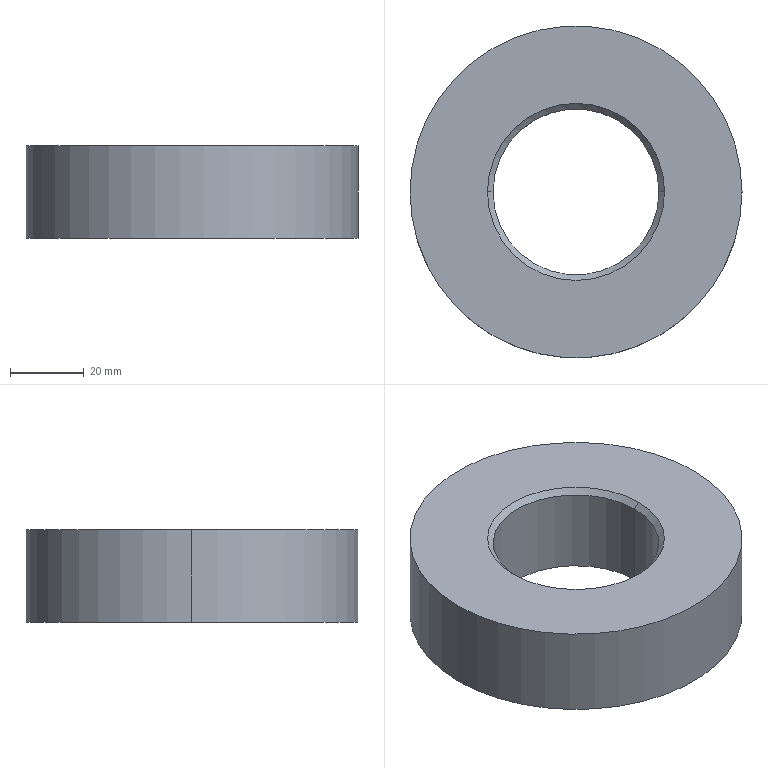Component | SolidWorks | BearingNew-1 | 1 solid | 8 faces | box 90 x 90 x 25 mm | volume 119120 mm3 | cylinder 4 | cone 2 | plane 2 | commonest cylinder face diameters 45 x2 90 x2
build123d program:
from build123d import *

# Parameters (mm, degrees)
SKETCH1_R           = 45
SKETCH1_R_2         = 22.5
BOSS_EXTRUDE1_DEPTH = 25
CHAMFER1_SIZE       = 1.5


with BuildPart() as part:
    # Sketch1 → Boss-Extrude1 (new body)
    with BuildSketch(Plane(origin=(0, 0, 0), x_dir=(0, 0, -1), z_dir=(1, 0, 0))):
        Circle(SKETCH1_R)
        Circle(SKETCH1_R_2, mode=Mode.SUBTRACT)
    extrude(amount=BOSS_EXTRUDE1_DEPTH)

    # Chamfer1
    chamfer1_edges = [part.edges().sort_by_distance(p)[0] for p in [
        (25, 0, 22.5),
    ]]
    chamfer(chamfer1_edges, length=CHAMFER1_SIZE)


solid = part.part

# Placed as in the assembly
solid = solid.moved(Location((35.733, 15.31, -0.5001), (0, -90, 0)))
STEP:
#1=COLOUR_RGB('',0.7922,0.8196,0.9333);
#2=FILL_AREA_STYLE_COLOUR('',#1);
#3=FILL_AREA_STYLE('',(#2));
#4=SURFACE_STYLE_FILL_AREA(#3);
#5=SURFACE_SIDE_STYLE('',(#4));
#6=SURFACE_STYLE_USAGE(.BOTH.,#5);
#7=PRESENTATION_STYLE_ASSIGNMENT((#6));
#8=CARTESIAN_POINT('',(0.521,0.6028,0.9055));
#9=VERTEX_POINT('',#8);
#10=CARTESIAN_POINT('',(2.293,0.6028,0.9055));
#11=VERTEX_POINT('',#10);
#12=CARTESIAN_POINT('',(1.407,0.6028,0.9055));
#13=DIRECTION('',(0.,-0.,1.));
#14=DIRECTION('',(1.,-0.,0.));
#15=AXIS2_PLACEMENT_3D('',#12,#13,#14);
#16=CIRCLE('',#15,0.8858);
#17=EDGE_CURVE('',#9,#11,#16,.T.);
#18=ORIENTED_EDGE('',*,*,#17,.F.);
#19=CARTESIAN_POINT('',(0.4619,0.6028,0.9646));
#20=VERTEX_POINT('',#19);
#21=CARTESIAN_POINT('',(0.521,0.6028,0.9055));
#22=DIRECTION('',(-0.7071,0.,0.7071));
#23=VECTOR('',#22,39.37);
#24=LINE('',#21,#23);
#25=EDGE_CURVE('',#9,#20,#24,.T.);
#26=ORIENTED_EDGE('',*,*,#25,.T.);
#27=CARTESIAN_POINT('',(2.352,0.6028,0.9646));
#28=VERTEX_POINT('',#27);
#29=CARTESIAN_POINT('',(1.407,0.6028,0.9646));
#30=DIRECTION('',(0.,0.,-1.));
#31=DIRECTION('',(1.,-0.,0.));
#32=AXIS2_PLACEMENT_3D('',#29,#30,#31);
#33=CIRCLE('',#32,0.9449);
#34=EDGE_CURVE('',#28,#20,#33,.T.);
#35=ORIENTED_EDGE('',*,*,#34,.F.);
#36=CARTESIAN_POINT('',(2.293,0.6028,0.9055));
#37=DIRECTION('',(0.7071,-0.,0.7071));
#38=VECTOR('',#37,39.37);
#39=LINE('',#36,#38);
#40=EDGE_CURVE('',#11,#28,#39,.T.);
#41=ORIENTED_EDGE('',*,*,#40,.F.);
#42=EDGE_LOOP('',(#18,#26,#35,#41));
#43=FACE_OUTER_BOUND('',#42,.T.);
#44=CARTESIAN_POINT('',(1.407,0.6028,0.9055));
#45=DIRECTION('',(0.,-0.,1.));
#46=DIRECTION('',(1.,-0.,0.));
#47=AXIS2_PLACEMENT_3D('',#44,#45,#46);
#48=CONICAL_SURFACE('',#47,0.8858,0.7854);
#49=ADVANCED_FACE('',(#43),#48,.F.);
#50=ORIENTED_EDGE('',*,*,#17,.T.);
#51=CARTESIAN_POINT('',(2.293,0.6028,-0.01969));
#52=VERTEX_POINT('',#51);
#53=CARTESIAN_POINT('',(2.293,0.6028,0.9646));
#54=DIRECTION('',(0.,0.,-1.));
#55=VECTOR('',#54,39.37);
#56=LINE('',#53,#55);
#57=EDGE_CURVE('',#11,#52,#56,.T.);
#58=ORIENTED_EDGE('',*,*,#57,.T.);
#59=CARTESIAN_POINT('',(0.521,0.6028,-0.01969));
#60=VERTEX_POINT('',#59);
#61=CARTESIAN_POINT('',(1.407,0.6028,-0.01969));
#62=DIRECTION('',(0.,-0.,1.));
#63=DIRECTION('',(1.,-0.,0.));
#64=AXIS2_PLACEMENT_3D('',#61,#62,#63);
#65=CIRCLE('',#64,0.8858);
#66=EDGE_CURVE('',#60,#52,#65,.T.);
#67=ORIENTED_EDGE('',*,*,#66,.F.);
#68=CARTESIAN_POINT('',(0.521,0.6028,0.9646));
#69=DIRECTION('',(0.,0.,-1.));
#70=VECTOR('',#69,39.37);
#71=LINE('',#68,#70);
#72=EDGE_CURVE('',#9,#60,#71,.T.);
#73=ORIENTED_EDGE('',*,*,#72,.F.);
#74=EDGE_LOOP('',(#50,#58,#67,#73));
#75=FACE_OUTER_BOUND('',#74,.T.);
#76=CARTESIAN_POINT('',(1.407,0.6028,0.9646));
#77=DIRECTION('',(0.,0.,-1.));
#78=DIRECTION('',(-1.,0.,0.));
#79=AXIS2_PLACEMENT_3D('',#76,#77,#78);
#80=CYLINDRICAL_SURFACE('',#79,0.8858);
#81=ADVANCED_FACE('',(#75),#80,.F.);
#82=CARTESIAN_POINT('',(3.178,0.6028,0.9646));
#83=VERTEX_POINT('',#82);
#84=CARTESIAN_POINT('',(-0.3649,0.6028,0.9646));
#85=VERTEX_POINT('',#84);
#86=CARTESIAN_POINT('',(1.407,0.6028,0.9646));
#87=DIRECTION('',(0.,-0.,1.));
#88=DIRECTION('',(1.,-0.,0.));
#89=AXIS2_PLACEMENT_3D('',#86,#87,#88);
#90=CIRCLE('',#89,1.772);
#91=EDGE_CURVE('',#83,#85,#90,.T.);
#92=ORIENTED_EDGE('',*,*,#91,.F.);
#93=CARTESIAN_POINT('',(3.178,0.6028,-0.01969));
#94=VERTEX_POINT('',#93);
#95=CARTESIAN_POINT('',(3.178,0.6028,0.9646));
#96=DIRECTION('',(0.,0.,-1.));
#97=VECTOR('',#96,39.37);
#98=LINE('',#95,#97);
#99=EDGE_CURVE('',#83,#94,#98,.T.);
#100=ORIENTED_EDGE('',*,*,#99,.T.);
#101=CARTESIAN_POINT('',(-0.3649,0.6028,-0.01969));
#102=VERTEX_POINT('',#101);
#103=CARTESIAN_POINT('',(1.407,0.6028,-0.01969));
#104=DIRECTION('',(0.,-0.,1.));
#105=DIRECTION('',(1.,-0.,0.));
#106=AXIS2_PLACEMENT_3D('',#103,#104,#105);
#107=CIRCLE('',#106,1.772);
#108=EDGE_CURVE('',#94,#102,#107,.T.);
#109=ORIENTED_EDGE('',*,*,#108,.T.);
#110=CARTESIAN_POINT('',(-0.3649,0.6028,0.9646));
#111=DIRECTION('',(0.,0.,-1.));
#112=VECTOR('',#111,39.37);
#113=LINE('',#110,#112);
#114=EDGE_CURVE('',#85,#102,#113,.T.);
#115=ORIENTED_EDGE('',*,*,#114,.F.);
#116=EDGE_LOOP('',(#92,#100,#109,#115));
#117=FACE_OUTER_BOUND('',#116,.T.);
#118=CARTESIAN_POINT('',(1.407,0.6028,0.9646));
#119=DIRECTION('',(0.,0.,-1.));
#120=DIRECTION('',(-1.,0.,0.));
#121=AXIS2_PLACEMENT_3D('',#118,#119,#120);
#122=CYLINDRICAL_SURFACE('',#121,1.772);
#123=ADVANCED_FACE('',(#117),#122,.T.);
#124=ORIENTED_EDGE('',*,*,#34,.T.);
#125=CARTESIAN_POINT('',(1.407,0.6028,0.9646));
#126=DIRECTION('',(0.,0.,-1.));
#127=DIRECTION('',(1.,-0.,0.));
#128=AXIS2_PLACEMENT_3D('',#125,#126,#127);
#129=CIRCLE('',#128,0.9449);
#130=EDGE_CURVE('',#20,#28,#129,.T.);
#131=ORIENTED_EDGE('',*,*,#130,.T.);
#132=EDGE_LOOP('',(#124,#131));
#133=FACE_BOUND('',#132,.T.);
#134=CARTESIAN_POINT('',(1.407,0.6028,0.9646));
#135=DIRECTION('',(0.,-0.,1.));
#136=DIRECTION('',(1.,-0.,0.));
#137=AXIS2_PLACEMENT_3D('',#134,#135,#136);
#138=CIRCLE('',#137,1.772);
#139=EDGE_CURVE('',#85,#83,#138,.T.);
#140=ORIENTED_EDGE('',*,*,#139,.T.);
#141=ORIENTED_EDGE('',*,*,#91,.T.);
#142=EDGE_LOOP('',(#140,#141));
#143=FACE_OUTER_BOUND('',#142,.T.);
#144=CARTESIAN_POINT('',(1.407,0.6028,0.9646));
#145=DIRECTION('',(-0.,-0.,1.));
#146=DIRECTION('',(1.,-0.,-0.));
#147=AXIS2_PLACEMENT_3D('',#144,#145,#146);
#148=PLANE('',#147);
#149=ADVANCED_FACE('',(#133,#143),#148,.T.);
#150=CARTESIAN_POINT('',(1.407,0.6028,-0.01969));
#151=DIRECTION('',(0.,-0.,1.));
#152=DIRECTION('',(1.,-0.,0.));
#153=AXIS2_PLACEMENT_3D('',#150,#151,#152);
#154=CIRCLE('',#153,1.772);
#155=EDGE_CURVE('',#102,#94,#154,.T.);
#156=ORIENTED_EDGE('',*,*,#155,.F.);
#157=ORIENTED_EDGE('',*,*,#108,.F.);
#158=EDGE_LOOP('',(#156,#157));
#159=FACE_OUTER_BOUND('',#158,.T.);
#160=ORIENTED_EDGE('',*,*,#66,.T.);
#161=CARTESIAN_POINT('',(1.407,0.6028,-0.01969));
#162=DIRECTION('',(0.,-0.,1.));
#163=DIRECTION('',(1.,-0.,0.));
#164=AXIS2_PLACEMENT_3D('',#161,#162,#163);
#165=CIRCLE('',#164,0.8858);
#166=EDGE_CURVE('',#52,#60,#165,.T.);
#167=ORIENTED_EDGE('',*,*,#166,.T.);
#168=EDGE_LOOP('',(#160,#167));
#169=FACE_BOUND('',#168,.T.);
#170=CARTESIAN_POINT('',(1.407,0.6028,-0.01969));
#171=DIRECTION('',(-0.,-0.,1.));
#172=DIRECTION('',(1.,-0.,-0.));
#173=AXIS2_PLACEMENT_3D('',#170,#171,#172);
#174=PLANE('',#173);
#175=ADVANCED_FACE('',(#159,#169),#174,.F.);
#176=ORIENTED_EDGE('',*,*,#99,.F.);
#177=ORIENTED_EDGE('',*,*,#139,.F.);
#178=ORIENTED_EDGE('',*,*,#114,.T.);
#179=ORIENTED_EDGE('',*,*,#155,.T.);
#180=EDGE_LOOP('',(#176,#177,#178,#179));
#181=FACE_OUTER_BOUND('',#180,.T.);
#182=CARTESIAN_POINT('',(1.407,0.6028,0.9646));
#183=DIRECTION('',(0.,0.,-1.));
#184=DIRECTION('',(-1.,0.,0.));
#185=AXIS2_PLACEMENT_3D('',#182,#183,#184);
#186=CYLINDRICAL_SURFACE('',#185,1.772);
#187=ADVANCED_FACE('',(#181),#186,.T.);
#188=ORIENTED_EDGE('',*,*,#57,.F.);
#189=CARTESIAN_POINT('',(1.407,0.6028,0.9055));
#190=DIRECTION('',(0.,-0.,1.));
#191=DIRECTION('',(1.,-0.,0.));
#192=AXIS2_PLACEMENT_3D('',#189,#190,#191);
#193=CIRCLE('',#192,0.8858);
#194=EDGE_CURVE('',#11,#9,#193,.T.);
#195=ORIENTED_EDGE('',*,*,#194,.T.);
#196=ORIENTED_EDGE('',*,*,#72,.T.);
#197=ORIENTED_EDGE('',*,*,#166,.F.);
#198=EDGE_LOOP('',(#188,#195,#196,#197));
#199=FACE_OUTER_BOUND('',#198,.T.);
#200=CARTESIAN_POINT('',(1.407,0.6028,0.9646));
#201=DIRECTION('',(0.,0.,-1.));
#202=DIRECTION('',(-1.,0.,0.));
#203=AXIS2_PLACEMENT_3D('',#200,#201,#202);
#204=CYLINDRICAL_SURFACE('',#203,0.8858);
#205=ADVANCED_FACE('',(#199),#204,.F.);
#206=ORIENTED_EDGE('',*,*,#25,.F.);
#207=ORIENTED_EDGE('',*,*,#194,.F.);
#208=ORIENTED_EDGE('',*,*,#40,.T.);
#209=ORIENTED_EDGE('',*,*,#130,.F.);
#210=EDGE_LOOP('',(#206,#207,#208,#209));
#211=FACE_OUTER_BOUND('',#210,.T.);
#212=CARTESIAN_POINT('',(1.407,0.6028,0.9055));
#213=DIRECTION('',(0.,-0.,1.));
#214=DIRECTION('',(1.,-0.,0.));
#215=AXIS2_PLACEMENT_3D('',#212,#213,#214);
#216=CONICAL_SURFACE('',#215,0.8858,0.7854);
#217=ADVANCED_FACE('',(#211),#216,.F.);
#218=CLOSED_SHELL('',(#49,#81,#123,#149,#175,#187,#205,#217));
#219=MANIFOLD_SOLID_BREP('',#218);
#220=STYLED_ITEM('',(#7),#219);
#221=(LENGTH_UNIT()NAMED_UNIT(*)SI_UNIT($,.METRE.));
#222=LENGTH_MEASURE_WITH_UNIT(LENGTH_MEASURE(0.0254),#221);
#223=DIMENSIONAL_EXPONENTS(1.,0.,0.,0.,0.,0.,0.);
#224=(CONVERSION_BASED_UNIT('',#222)LENGTH_UNIT()NAMED_UNIT(#223));
#225=UNCERTAINTY_MEASURE_WITH_UNIT(LENGTH_MEASURE(0.00001),#224,'','');
#226=(NAMED_UNIT(*)PLANE_ANGLE_UNIT()SI_UNIT($,.RADIAN.));
#227=(NAMED_UNIT(*)SI_UNIT($,.STERADIAN.)SOLID_ANGLE_UNIT());
#228=(GEOMETRIC_REPRESENTATION_CONTEXT(3)GLOBAL_UNCERTAINTY_ASSIGNED_CONTEXT((#225))GLOBAL_UNIT_ASSIGNED_CONTEXT((#224,#226,#227))REPRESENTATION_CONTEXT('',''));
#229=MECHANICAL_DESIGN_GEOMETRIC_PRESENTATION_REPRESENTATION('',(#220),#228);
#230=CARTESIAN_POINT('',(0.,0.,0.));
#231=DIRECTION('',(0.,0.,1.));
#232=DIRECTION('',(1.,0.,0.));
#233=AXIS2_PLACEMENT_3D('',#230,#231,#232);
#234=(LENGTH_UNIT()NAMED_UNIT(*)SI_UNIT($,.METRE.));
#235=LENGTH_MEASURE_WITH_UNIT(LENGTH_MEASURE(0.0254),#234);
#236=DIMENSIONAL_EXPONENTS(1.,0.,0.,0.,0.,0.,0.);
#237=(CONVERSION_BASED_UNIT('',#235)LENGTH_UNIT()NAMED_UNIT(#236));
#238=UNCERTAINTY_MEASURE_WITH_UNIT(LENGTH_MEASURE(0.00001),#237,'','');
#239=(NAMED_UNIT(*)PLANE_ANGLE_UNIT()SI_UNIT($,.RADIAN.));
#240=(NAMED_UNIT(*)SI_UNIT($,.STERADIAN.)SOLID_ANGLE_UNIT());
#241=(GEOMETRIC_REPRESENTATION_CONTEXT(3)GLOBAL_UNCERTAINTY_ASSIGNED_CONTEXT((#238))GLOBAL_UNIT_ASSIGNED_CONTEXT((#237,#239,#240))REPRESENTATION_CONTEXT('',''));
#242=ADVANCED_BREP_SHAPE_REPRESENTATION('',(#219,#233),#241);
#243=PRESENTATION_LAYER_ASSIGNMENT('','',(#220));